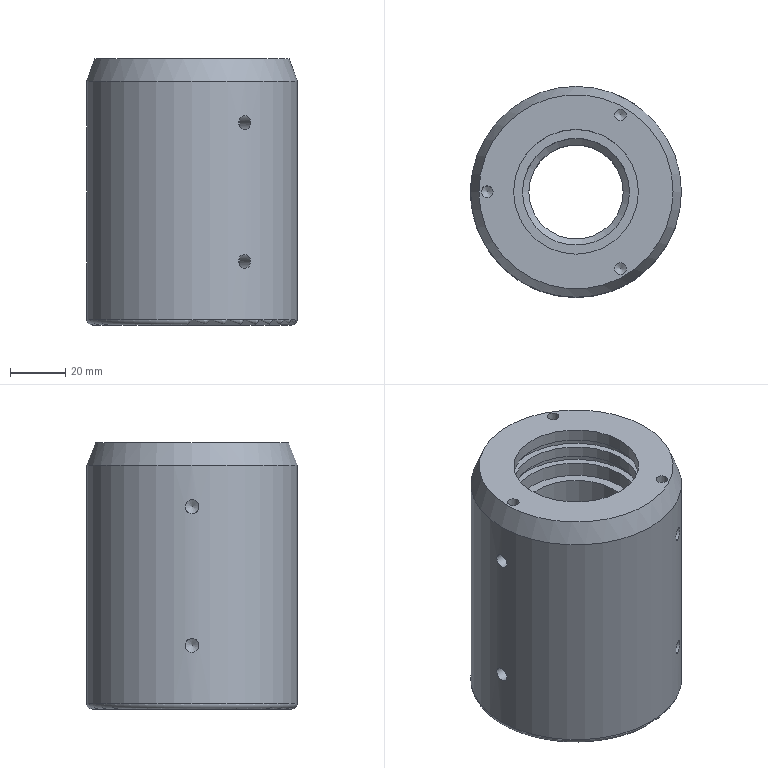Component | NX | CH3404_8-2 | 1 solid | 43 faces | volume 318411 mm3 | cylinder 20 | cone 14 | plane 7 | torus 2 | commonest cylinder face diameters 5 x9 45 x3 4.2 x3 49.6 x2 76 x1 34 x1 38.6 x1